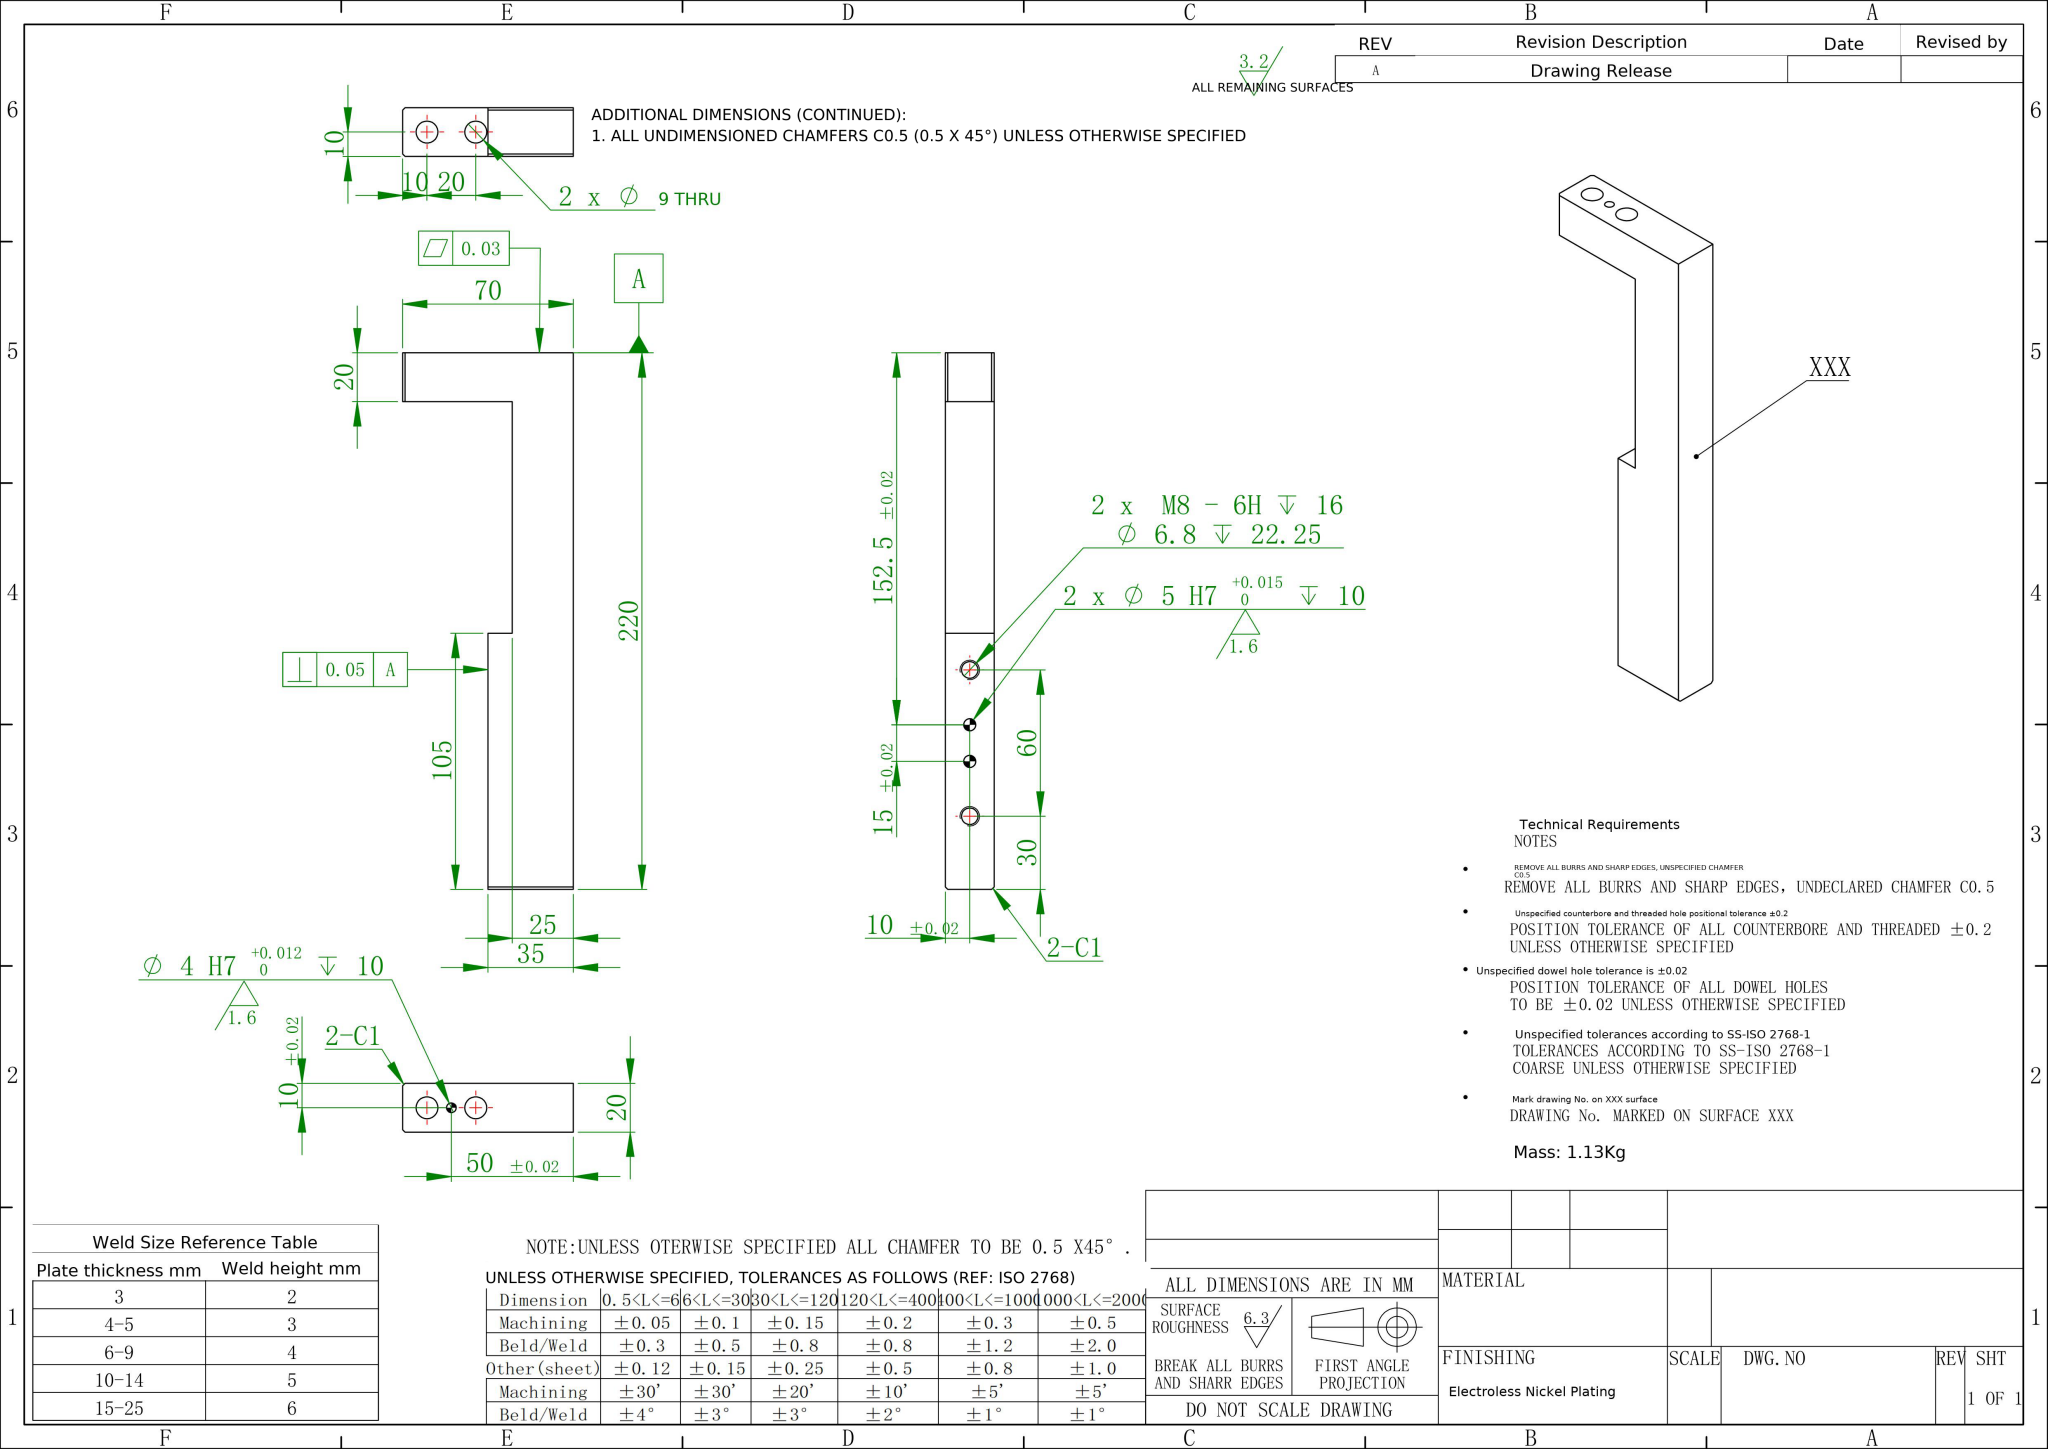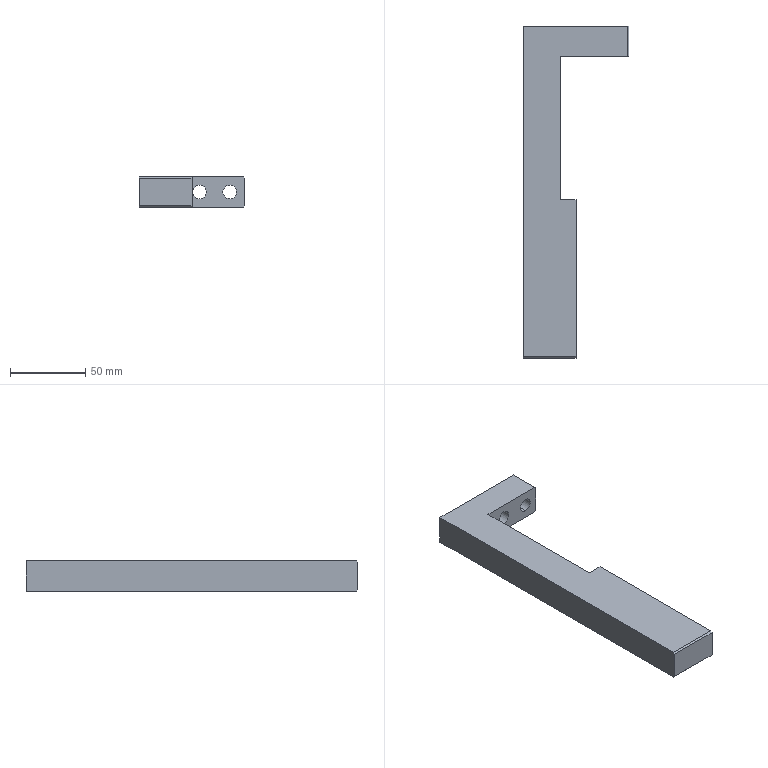Part | NX | mm | 1 solid | 38 faces | box 70 x 220 x 20 mm | volume 144192 mm3 | cylinder 14 | plane 14 | cone 10 | commonest cylinder face diameters 5 x4 6.8 x4 9 x4 4 x2